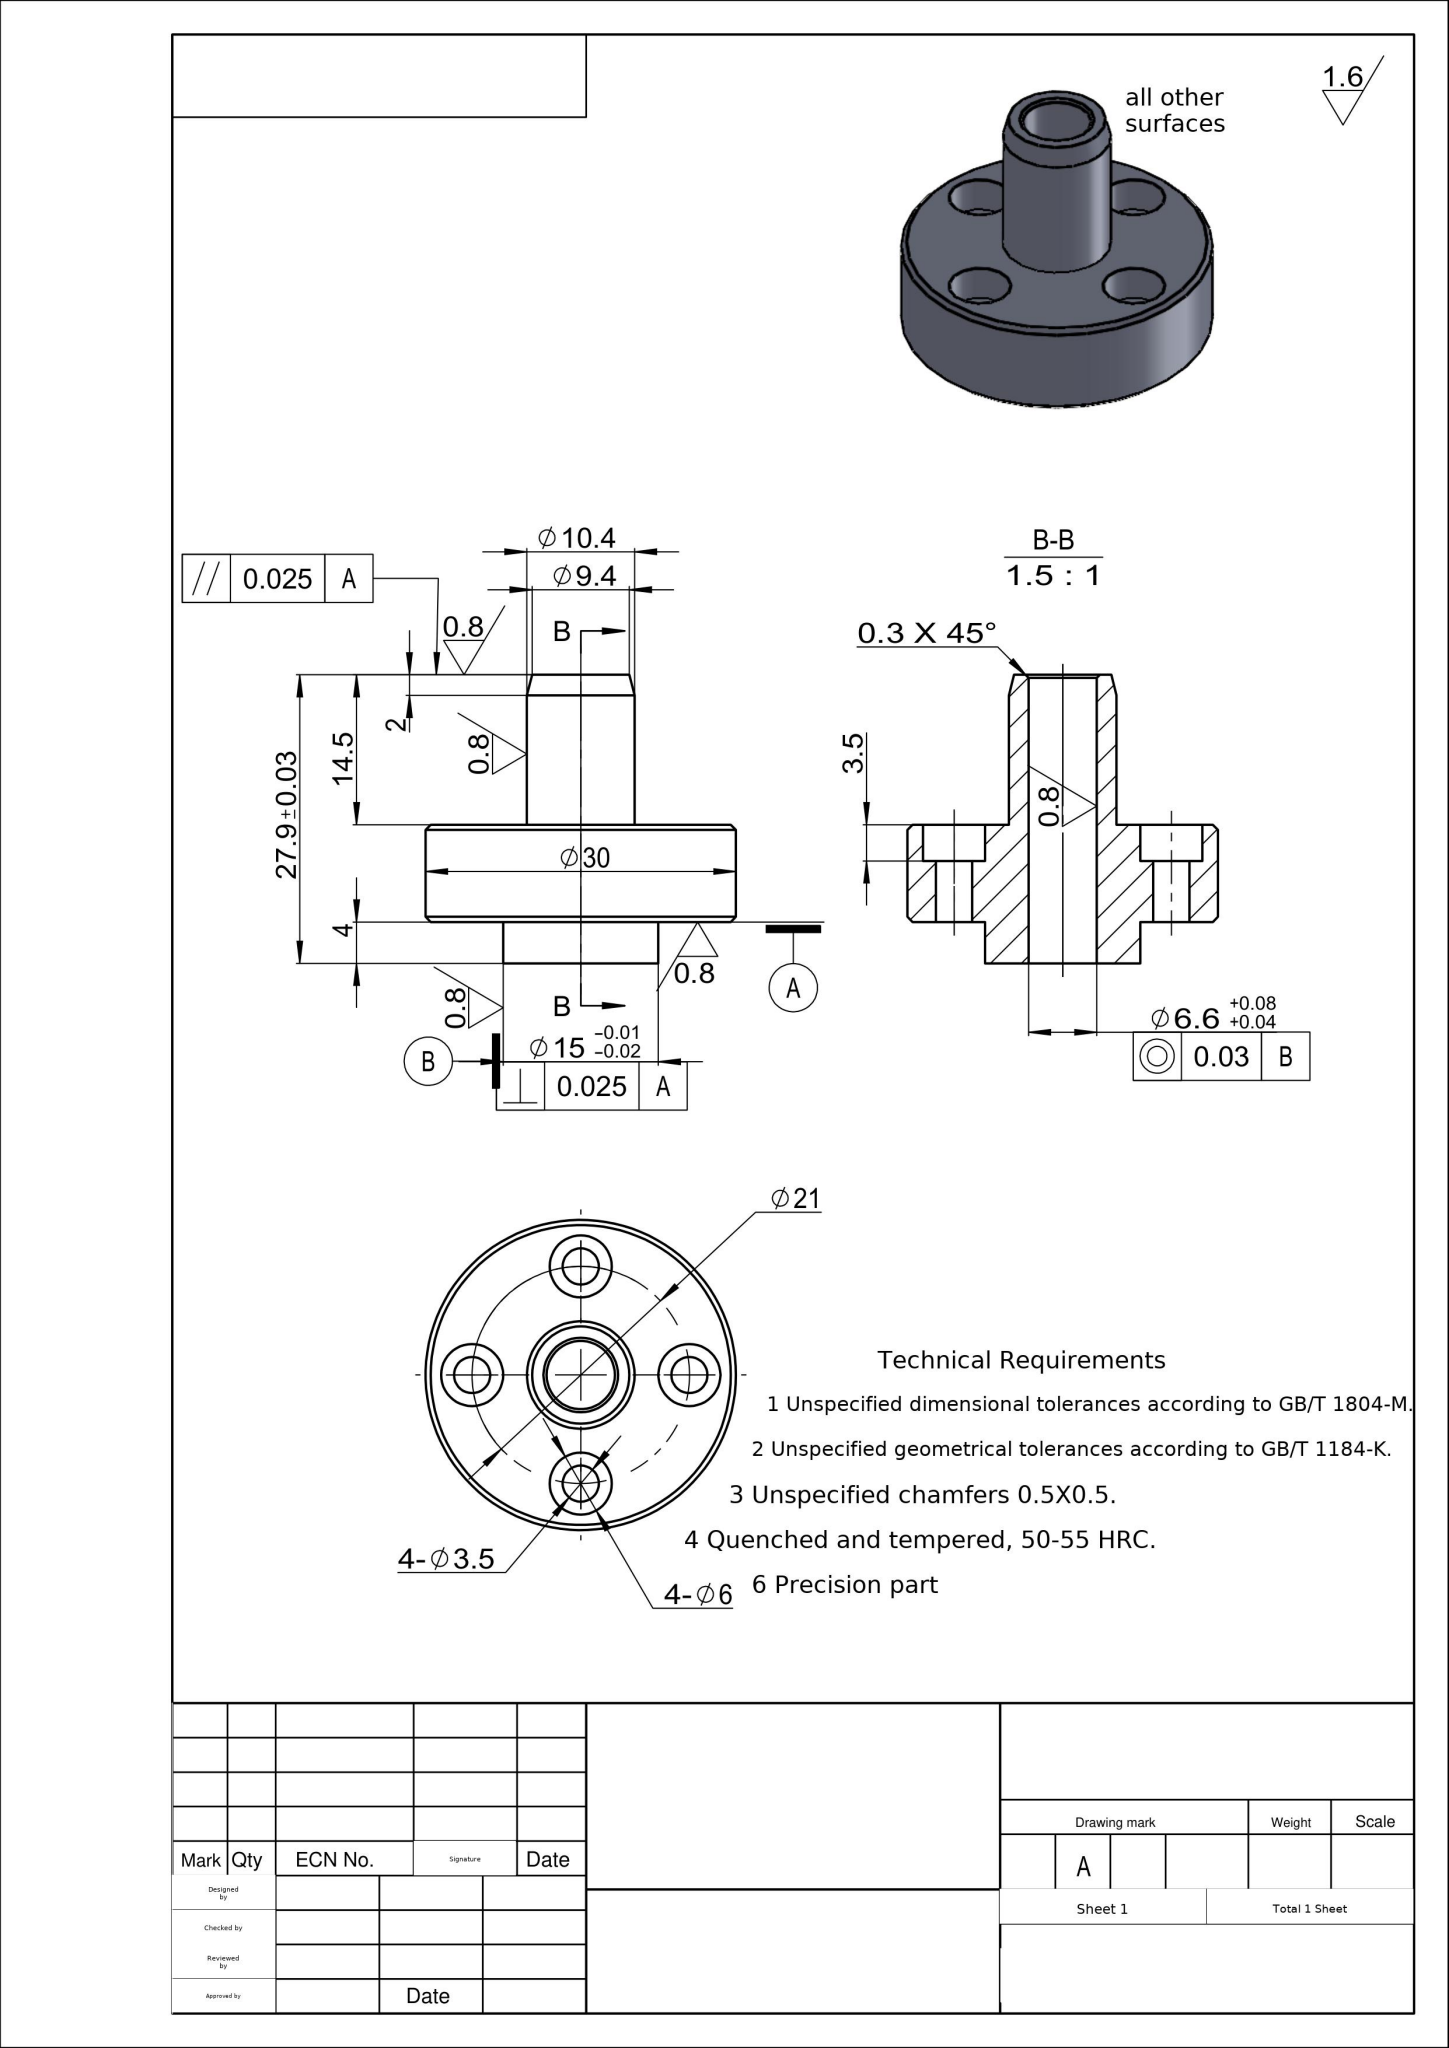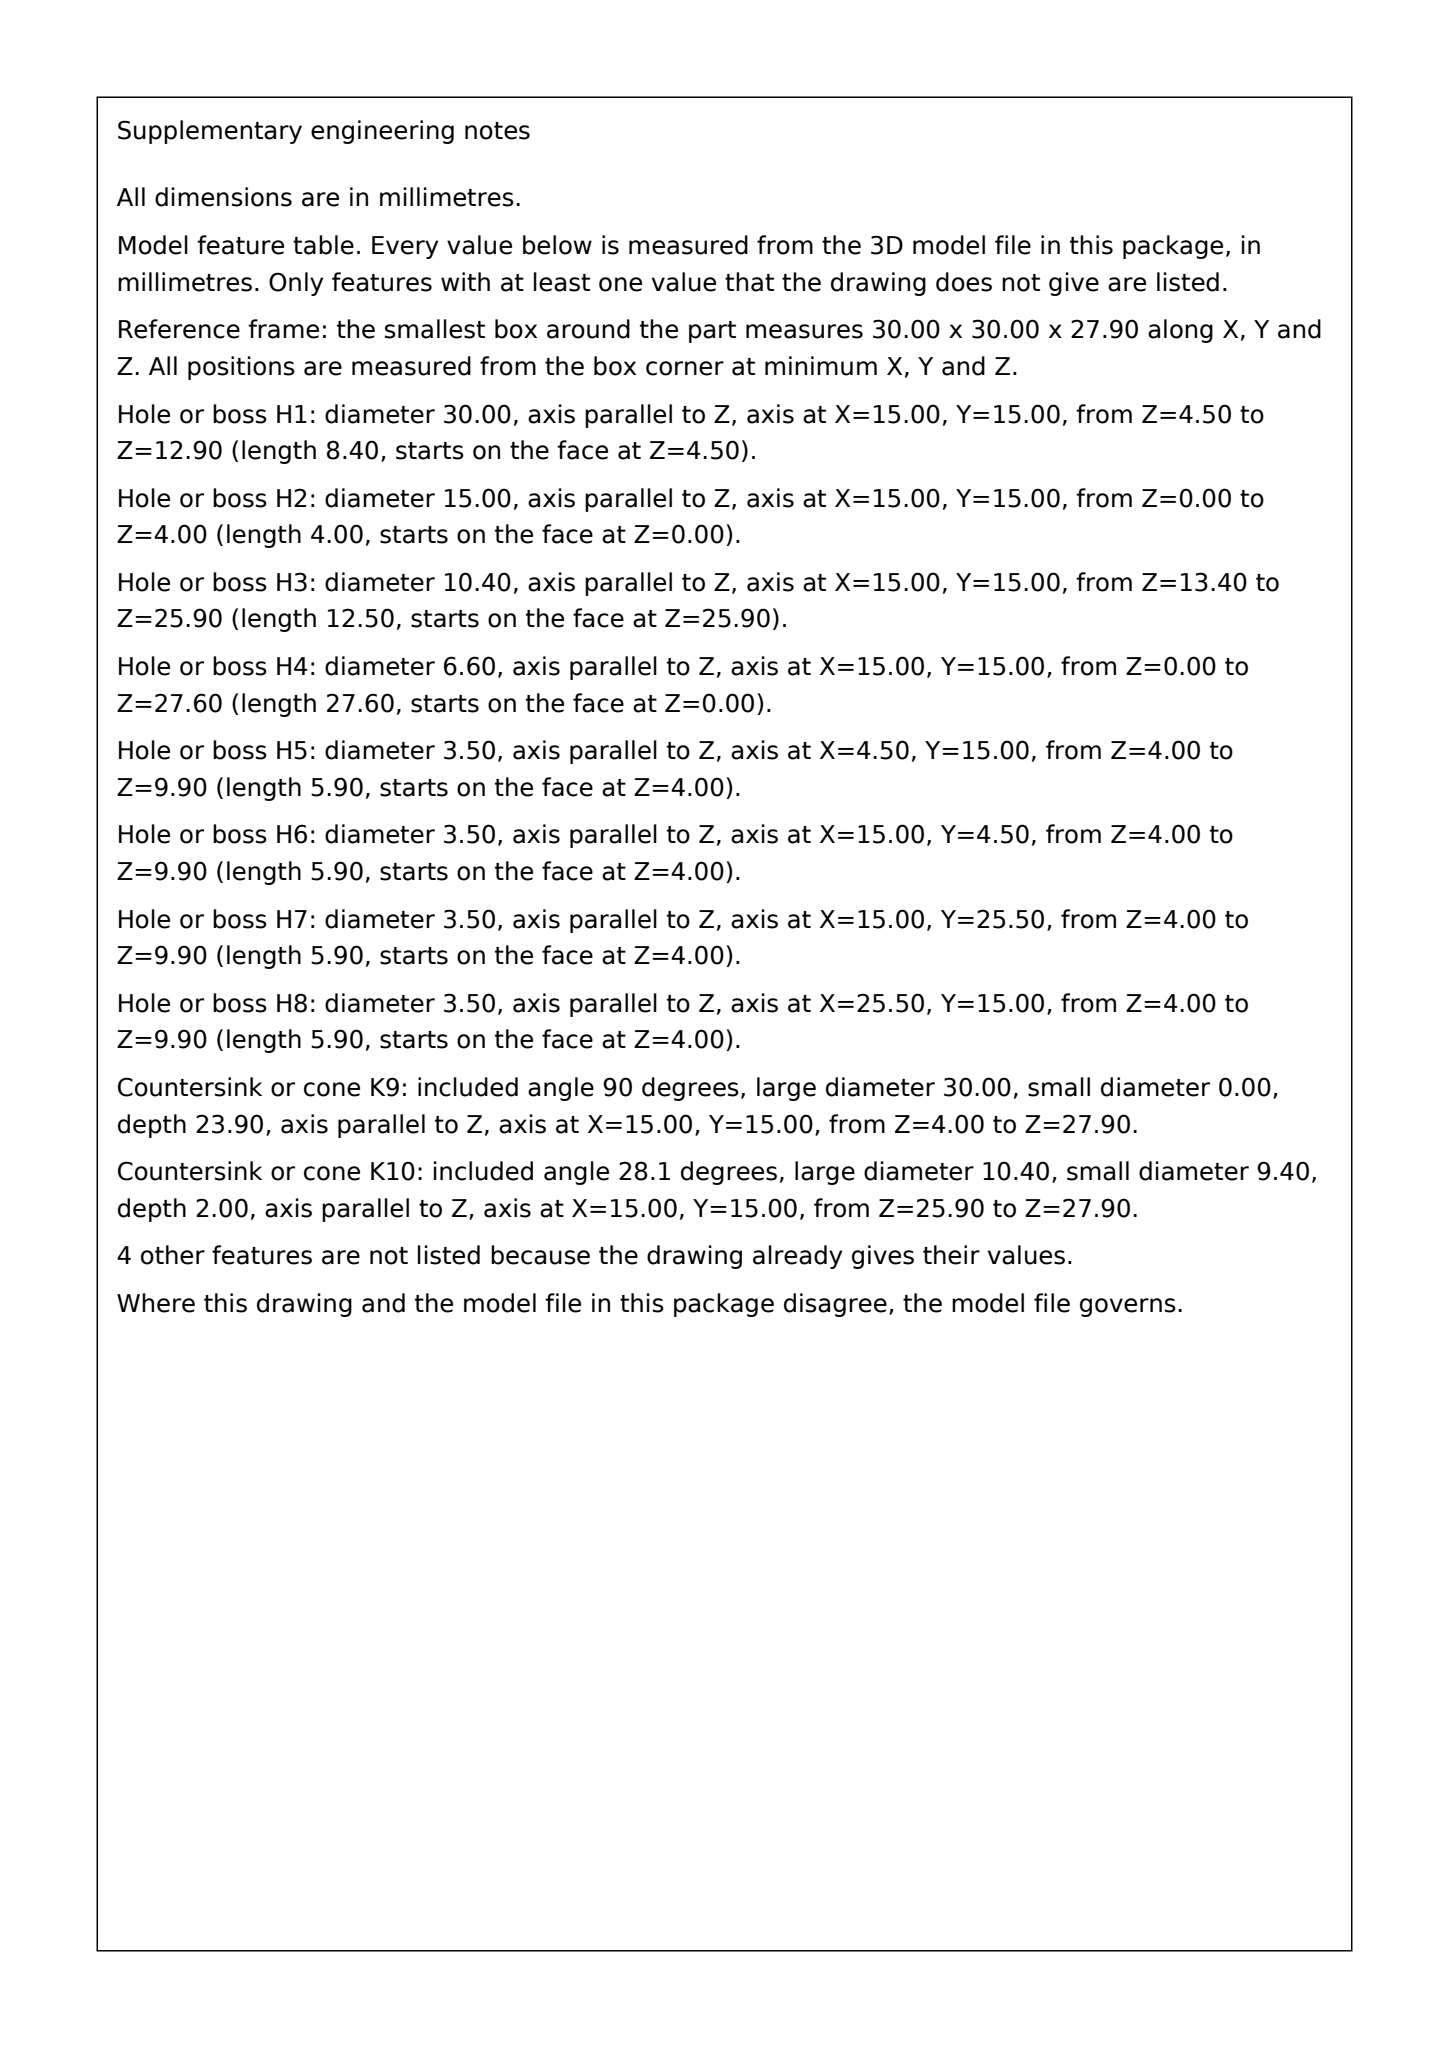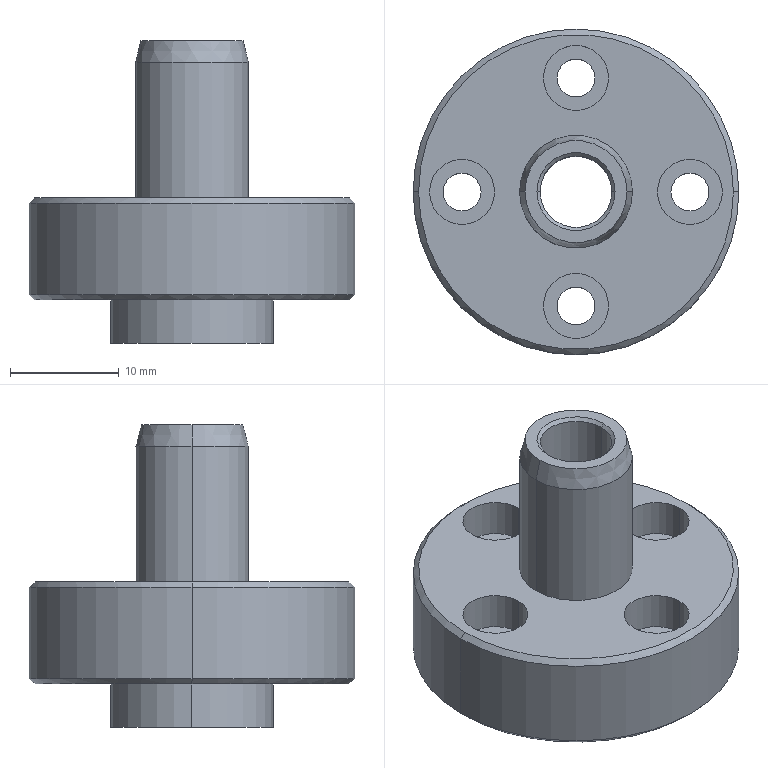Part | SolidWorks | mm | 1 solid | 40 faces | box 30 x 30 x 27.9 mm | volume 6966 mm3 | cylinder 24 | cone 8 | plane 8 | commonest cylinder face diameters 6 x8 3.5 x8 15 x2 6.6 x2 10.4 x2 30 x2
build123d program:
from build123d import *

# Parameters (mm, degrees)
SKETCH1_R           = 15
BOSS_EXTRUDE1_DEPTH = 9.4
SKETCH2_R           = 5.2
BOSS_EXTRUDE2_DEPTH = 14.5
SKETCH3_R           = 3.3
CUT_EXTRUDE1_DEPTH  = 100
SKETCH5_R           = 7.5
SKETCH5_R_2         = 3.3
BOSS_EXTRUDE3_DEPTH = 4
CHAMFER1_SIZE       = 0.5
SKETCH6_R           = 1.75
CUT_EXTRUDE2_DEPTH  = 26.695
SKETCH7_R           = 3
CUT_EXTRUDE3_DEPTH  = 3.5
CIRPATTERN1_COUNT   = 4
CHAMFER2_SIZE       = 0.3


with BuildPart() as part:
    # Sketch1 → Boss-Extrude1 (new body)
    with BuildSketch(Plane.XY):
        Circle(SKETCH1_R)
    extrude(amount=BOSS_EXTRUDE1_DEPTH)

    # Sketch2 → Boss-Extrude2 (add)
    with BuildSketch(Plane.XY.offset(9.4)):
        with Locations(Location((0, 0, 0), (0, 0, 180))):
            Circle(SKETCH2_R)
    extrude(amount=BOSS_EXTRUDE2_DEPTH)

    # Sketch3 → Cut-Extrude1 (cut)
    with BuildSketch(Plane.XY.offset(23.9)):
        Circle(SKETCH3_R)
    extrude(amount=-CUT_EXTRUDE1_DEPTH, mode=Mode.SUBTRACT)

    # Sketch4 → Cut-Revolve1 (revolve, cut)
    with BuildSketch(Plane(origin=(0, 0, 0), x_dir=(1, 0, 0), z_dir=(0, 1, 0)), mode=Mode.PRIVATE) as cut_revolve1_sk:
        Polygon((5.2, -23.9), (5.2, -21.9), (4.7, -23.9), align=None)
    revolve(cut_revolve1_sk.sketch.rotate(Axis((0, 0, 23.9), (0, 0, -1)), 180), axis=Axis((0, 0, 23.9), (0, 0, -1)), mode=Mode.SUBTRACT)

    # Sketch5 → Boss-Extrude3 (add)
    with BuildSketch(Plane(origin=(0, 0, 0), x_dir=(-1, 0, 0), z_dir=(0, 0, -1))):
        with Locations(Location((0, 0, 0), (0, 0, 180))):
            Circle(SKETCH5_R)
        with Locations(Location((0, 0, 0), (0, 0, 180))):
            Circle(SKETCH5_R_2, mode=Mode.SUBTRACT)
    extrude(amount=BOSS_EXTRUDE3_DEPTH)

    # Chamfer1
    chamfer1_edges = [part.edges().sort_by_distance(p)[0] for p in [
        (-15, 0, 0),
        (-15, 0, 9.4),
    ]]
    chamfer(chamfer1_edges, length=CHAMFER1_SIZE)

    # Sketch6 → Cut-Extrude2 (cut, through all)
    with BuildSketch(Plane.XY.offset(9.4)):
        with Locations((0, -10.5)):
            Circle(SKETCH6_R)
    cut_extrude2 = extrude(amount=-CUT_EXTRUDE2_DEPTH, mode=Mode.SUBTRACT)

    # Sketch7 → Cut-Extrude3 (cut)
    with BuildSketch(Plane.XY.offset(9.4)):
        with Locations((0, -10.5)):
            Circle(SKETCH7_R)
    cut_extrude3 = extrude(amount=-CUT_EXTRUDE3_DEPTH, mode=Mode.SUBTRACT)

    # CirPattern1: Cut-Extrude2, Cut-Extrude3 ×4 about axis
    cirpattern1_axis = Axis((0, 0, 0), (0, 0, 1))
    add([cut_extrude2.rotate(cirpattern1_axis, i * 360 / CIRPATTERN1_COUNT) for i in range(1, CIRPATTERN1_COUNT)], mode=Mode.SUBTRACT)
    add([cut_extrude3.rotate(cirpattern1_axis, i * 360 / CIRPATTERN1_COUNT) for i in range(1, CIRPATTERN1_COUNT)], mode=Mode.SUBTRACT)

    # Chamfer2
    chamfer2_edges = [part.edges().sort_by_distance(p)[0] for p in [
        (-3.3, 0, 23.9),
    ]]
    chamfer(chamfer2_edges, length=CHAMFER2_SIZE)


solid = part.part